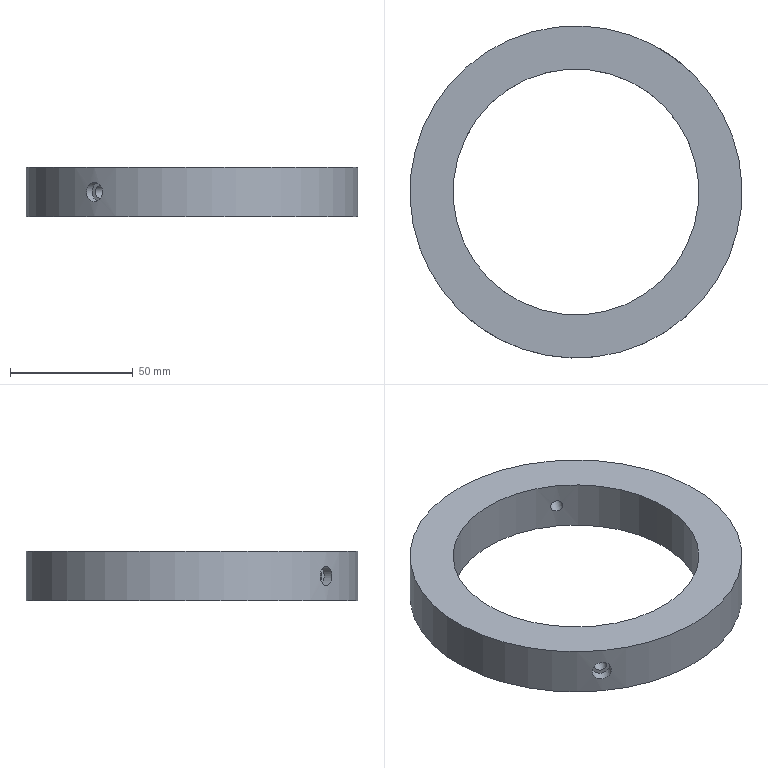Component | NX | CA6140-ZHUZHOU-JINYOUHUAN | 1 solid | 10 faces | volume 128271 mm3 | cylinder 6 | plane 4 | commonest cylinder face diameters 5 x2 8 x2 135 x1 100 x1